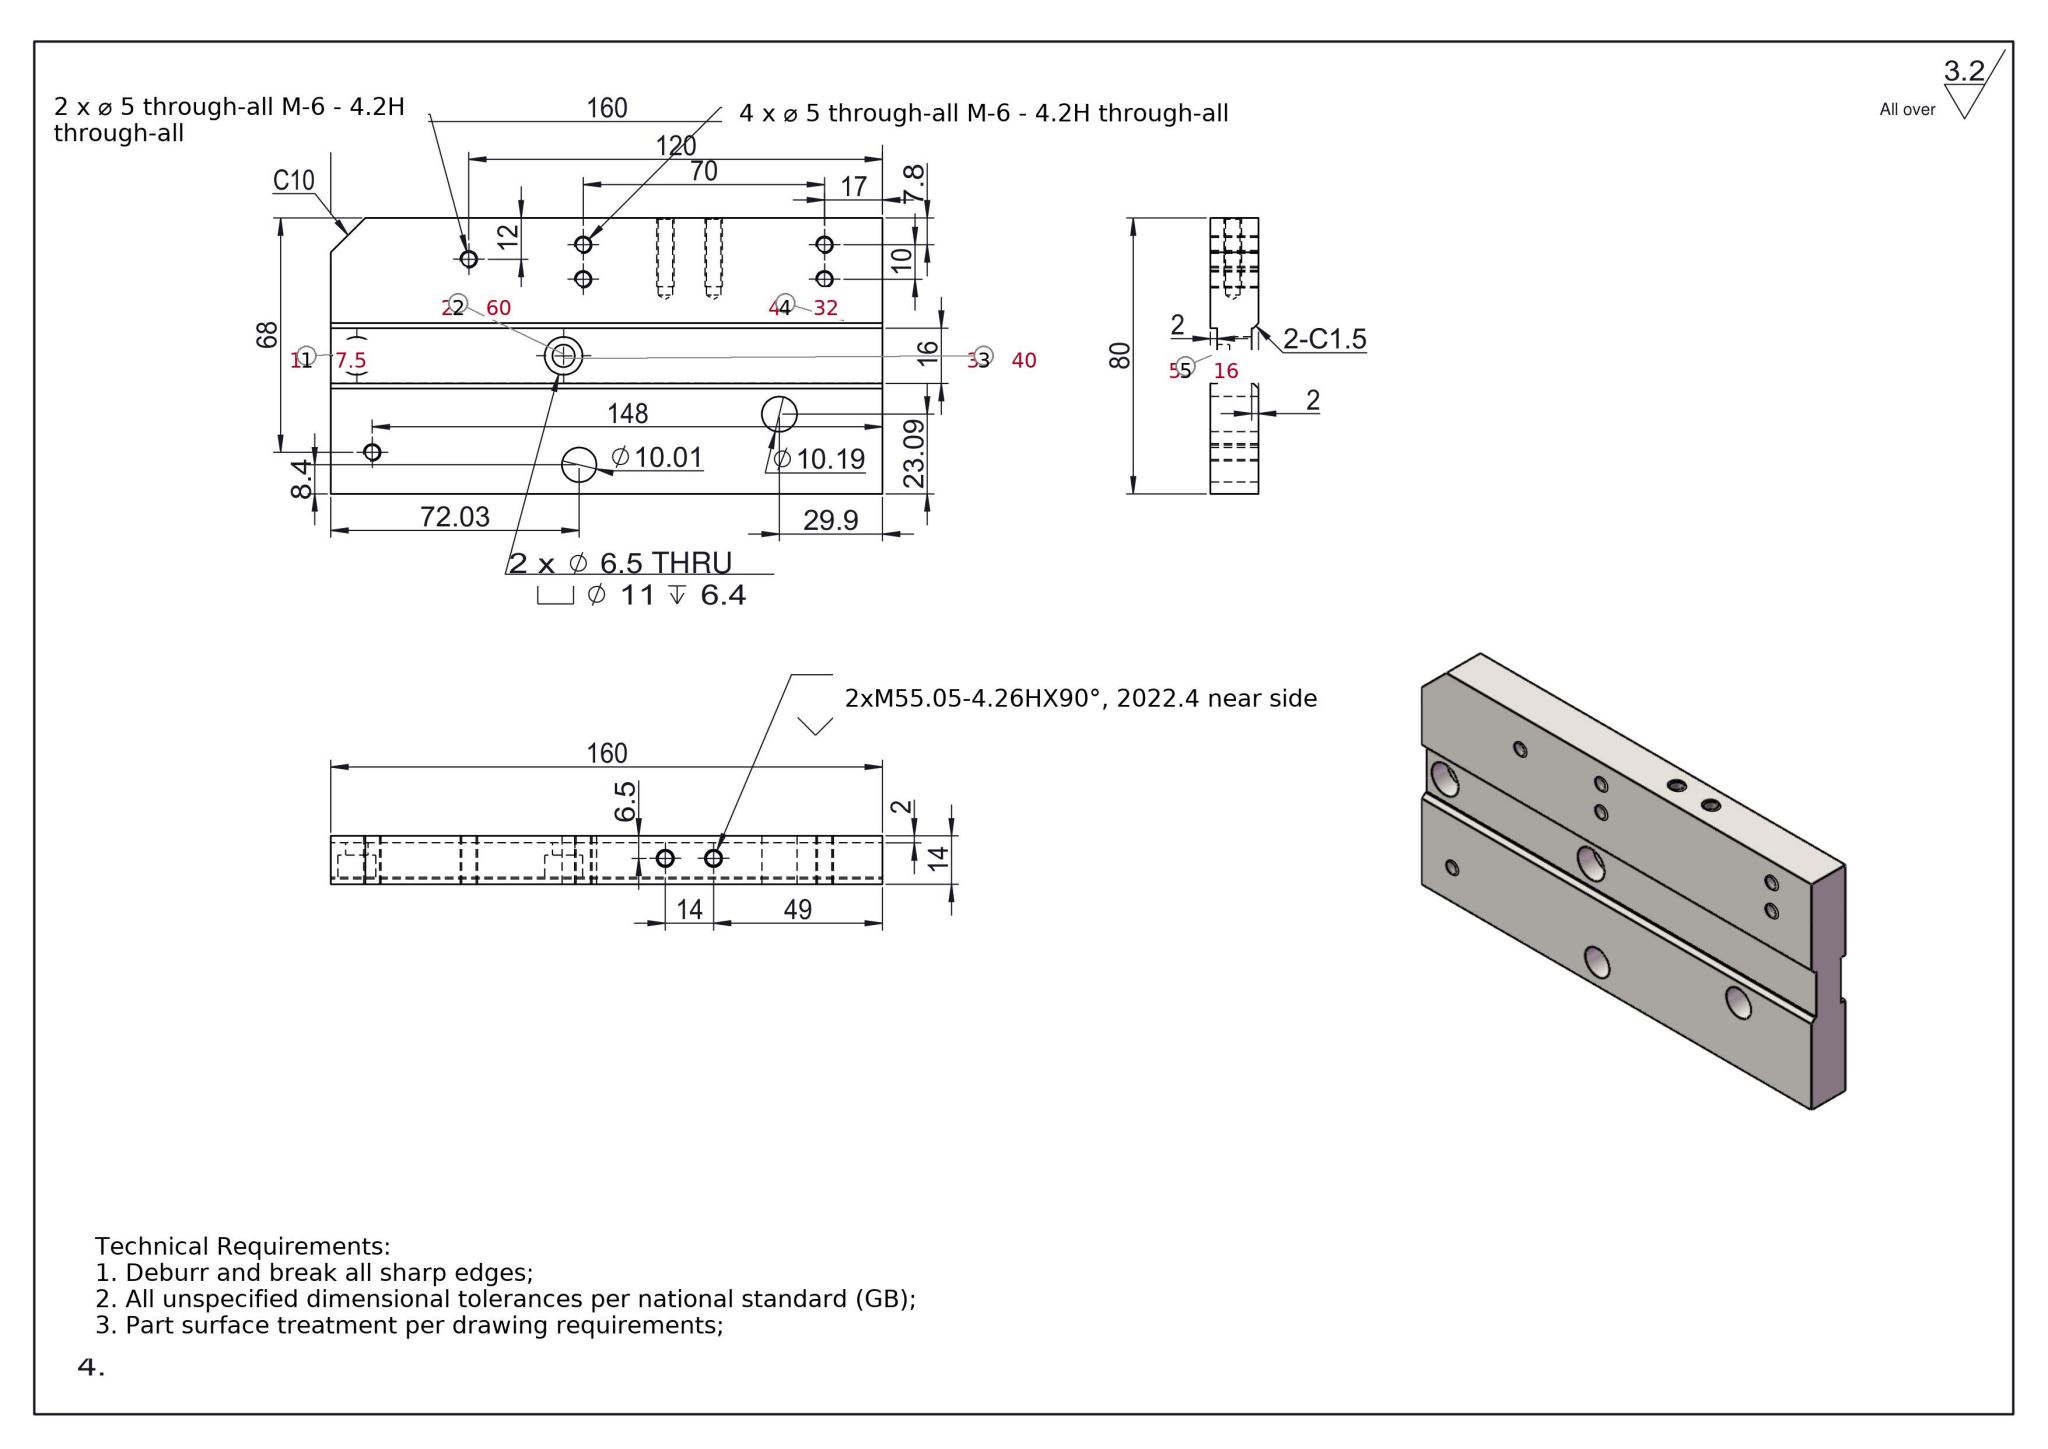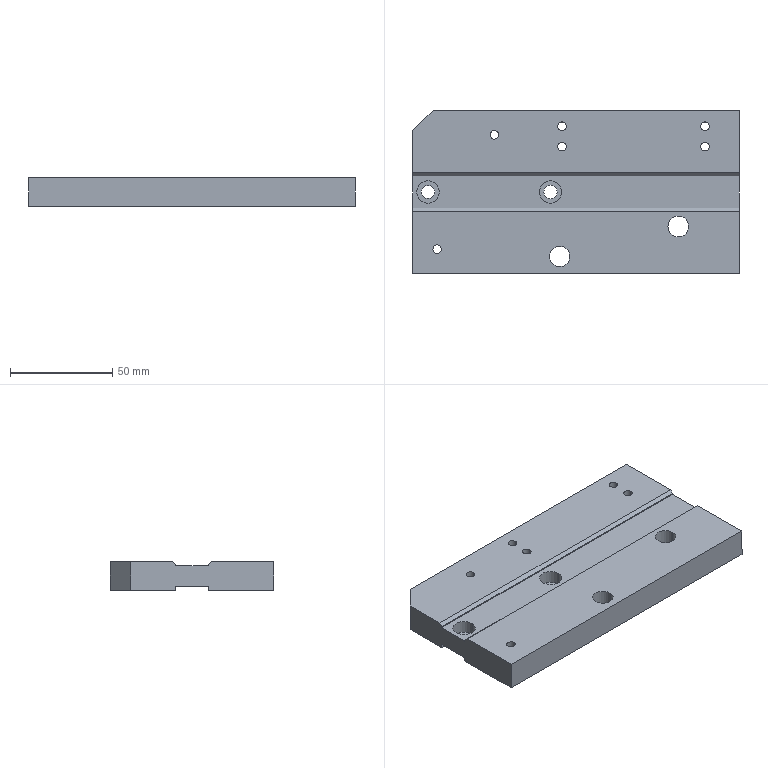Part | SolidWorks | mm | 1 solid | 55 faces | box 160 x 80 x 14 mm | volume 162407 mm3 | cylinder 28 | plane 19 | cone 8 | commonest cylinder face diameters 4.2 x16 11 x4 6.5 x4 10.194 x2 10.014 x2
build123d program:
from build123d import *

# Parameters (mm, degrees)
SKETCH1_W                                       = 160
SKETCH1_H                                       = 79.998
BOSS_EXTRUDE1_DEPTH                             = 12
SKETCH2_W                                       = 160
SKETCH2_H                                       = 32.031
SKETCH2_H_2                                     = 31.998
BOSS_EXTRUDE2_DEPTH                             = 2
SKETCH3_W                                       = 160
SKETCH3_H                                       = 16
CUT_EXTRUDE1_DEPTH                              = 2
CHAMFER1_SIZE                                   = 1.5
M5_TAPPED_HOLE1_D                               = 4.2
M5_TAPPED_HOLE1_DEPTH                           = 22.4
M5_TAPPED_HOLE1_CSINK_D                         = 5.05
M5_TAPPED_HOLE1_CSINK_ANGLE                     = 90
M5_TAPPED_HOLE1_TIP                             = 1.262
M6_HEX_SOCKET_HEAD_CAP_SCREW_CBORE1_D           = 6.5
M6_HEX_SOCKET_HEAD_CAP_SCREW_CBORE1_CBORE_D     = 11
M6_HEX_SOCKET_HEAD_CAP_SCREW_CBORE1_CBORE_DEPTH = 6.4
M5_TAPPED_HOLE2_D                               = 4.2
M5_TAPPED_HOLE3_D                               = 4.2
CHAMFER2_SIZE                                   = 10
SKETCH12_R                                      = 5.097
SKETCH12_R_2                                    = 5.007
CUT_EXTRUDE2_DEPTH                              = 80


with BuildPart() as part:
    # Sketch1 → Boss-Extrude1 (new body)
    with BuildSketch(Plane.XY):
        with Locations((80, -0.0008052)):
            Rectangle(SKETCH1_W, SKETCH1_H)
    extrude(amount=BOSS_EXTRUDE1_DEPTH)

    # Sketch2 → Boss-Extrude2 (add)
    with BuildSketch(Plane(origin=(0, 0, 0), x_dir=(-1, 0, 0), z_dir=(0, 0, -1))):
        with Locations((-80, -23.985)):
            Rectangle(SKETCH2_W, SKETCH2_H)
        with Locations((-80, 23.999)):
            Rectangle(SKETCH2_W, SKETCH2_H_2)
    extrude(amount=BOSS_EXTRUDE2_DEPTH)

    # Sketch3 → Cut-Extrude1 (cut)
    with BuildSketch(Plane.XY.offset(12)):
        with Locations((80, 0)):
            Rectangle(SKETCH3_W, SKETCH3_H)
    extrude(amount=-CUT_EXTRUDE1_DEPTH, mode=Mode.SUBTRACT)

    # Chamfer1
    chamfer1_edges = [part.edges().sort_by_distance(p)[0] for p in [
        (80, -8, 12),
        (80, 8, 12),
    ]]
    chamfer(chamfer1_edges, length=CHAMFER1_SIZE)

    # M5 Tapped Hole1
    with Locations(Plane(origin=(0, 39.998, 0), x_dir=(1, 0, 0), z_dir=(0, 1, 0))):
        with Locations((111, -4.5), (97, -4.5)):
            CounterSinkHole(M5_TAPPED_HOLE1_D / 2, M5_TAPPED_HOLE1_CSINK_D / 2, depth=M5_TAPPED_HOLE1_DEPTH, counter_sink_angle=M5_TAPPED_HOLE1_CSINK_ANGLE)
            with Locations((0, 0, -(M5_TAPPED_HOLE1_DEPTH + M5_TAPPED_HOLE1_TIP / 2))):  # 118° drill point
                Cone(0, M5_TAPPED_HOLE1_D / 2, M5_TAPPED_HOLE1_TIP, mode=Mode.SUBTRACT)

    # M6 Hex Socket Head Cap Screw CBORE1 (through all)
    with Locations(Plane.XY.offset(10)):
        with Locations((67.5, 0), (7.5, 0)):
            CounterBoreHole(M6_HEX_SOCKET_HEAD_CAP_SCREW_CBORE1_D / 2, M6_HEX_SOCKET_HEAD_CAP_SCREW_CBORE1_CBORE_D / 2, M6_HEX_SOCKET_HEAD_CAP_SCREW_CBORE1_CBORE_DEPTH)

    # M5 Tapped Hole2 (through all)
    with Locations(Plane.XY.offset(12)):
        with Locations((40, 27.998), (12, -28)):
            Hole(M5_TAPPED_HOLE2_D / 2)

    # M5 Tapped Hole3 (through all)
    with Locations(Plane.XY.offset(12)):
        with Locations((73.19, 32.199), (73.19, 22.199), (143.19, 32.199), (143.19, 22.199)):
            Hole(M5_TAPPED_HOLE3_D / 2)

    # Chamfer2
    chamfer2_edges = [part.edges().sort_by_distance(p)[0] for p in [
        (0, 39.998, 5),
    ]]
    chamfer(chamfer2_edges, length=CHAMFER2_SIZE)

    # Sketch12 → Cut-Extrude2 (cut)
    with BuildSketch(Plane.XY.offset(12)):
        with Locations((130.099, -16.907)):
            Circle(SKETCH12_R)
        with Locations((72.034, -31.6)):
            Circle(SKETCH12_R_2)
    extrude(amount=-CUT_EXTRUDE2_DEPTH, mode=Mode.SUBTRACT)


solid = part.part